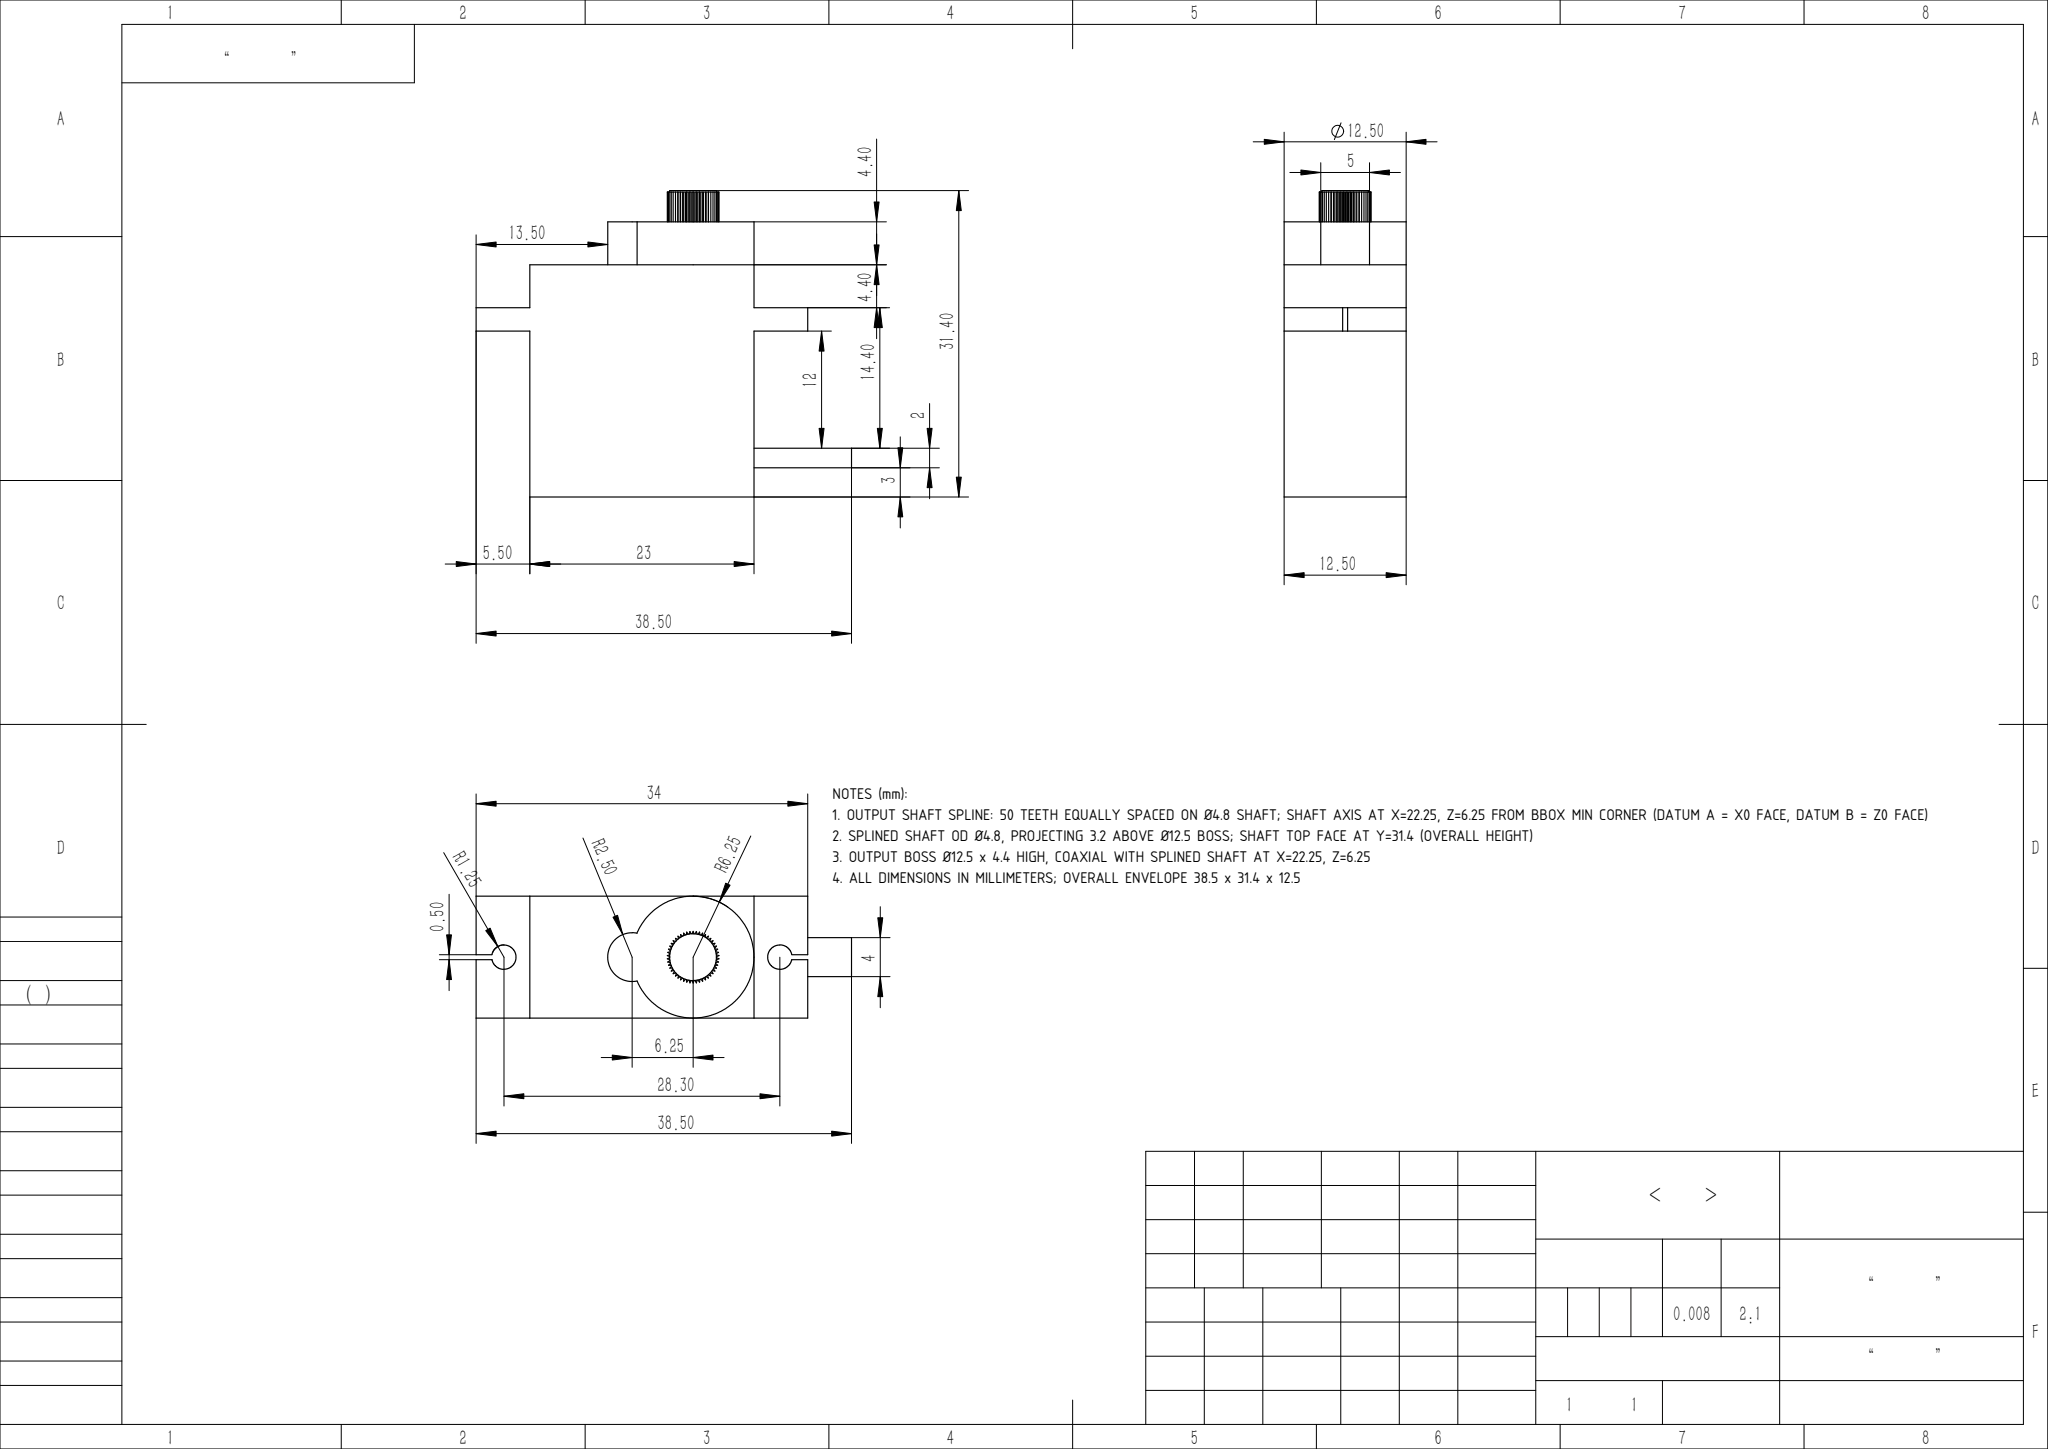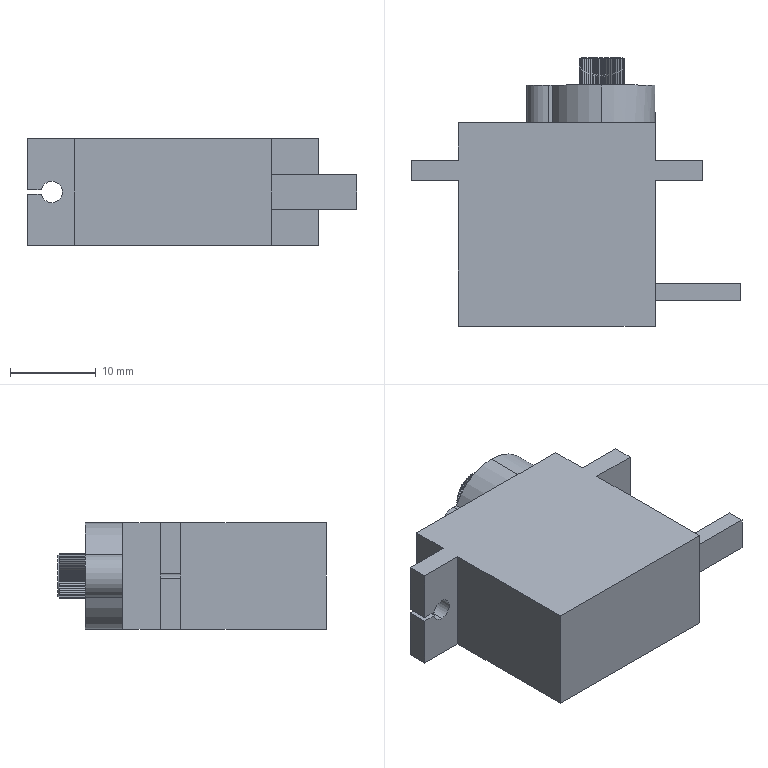Part | SolidWorks | mm | 1 solid | 193 faces | box 38.5 x 31.4 x 12.5 mm | volume 7874 mm3 | plane 179 | cylinder 14 | commonest cylinder face diameters 2.5 x6 5 x3 12.5 x3 4.8 x2
Drawing notes:
OUTPUT SHAFT SPLINE: 50 TEETH EQUALLY SPACED ON Ø4.8 SHAFT; SHAFT AXIS AT X=22.25, Z=6.25 FROM BBOX MIN CORNER (DATUM A = X0 FACE, DATUM B = Z0 FACE) | from the solid: axis_planes ["y",31.25]:count 50 (50 spline flats) with cylinder [4.8,"y",[22.25,null,6.25],3.2]
SPLINED SHAFT OD Ø4.8, PROJECTING 3.2 ABOVE Ø12.5 BOSS; SHAFT TOP FACE AT Y=31.4 (OVERALL HEIGHT) | from the solid: cylinder [4.8,"y",[22.25,null,6.25],3.2]; axis_plane ["y",31.4]; bbox_xyz Y=31.4
OUTPUT BOSS Ø12.5 x 4.4 HIGH, COAXIAL WITH SPLINED SHAFT AT X=22.25, Z=6.25 | from the solid: cylinder [12.5,"y",[22.25,null,6.25],4.4]
ALL DIMENSIONS IN MILLIMETERS; OVERALL ENVELOPE 38.5 x 31.4 x 12.5 | from the solid: bbox_xyz [38.5,31.4,12.5] (mm)